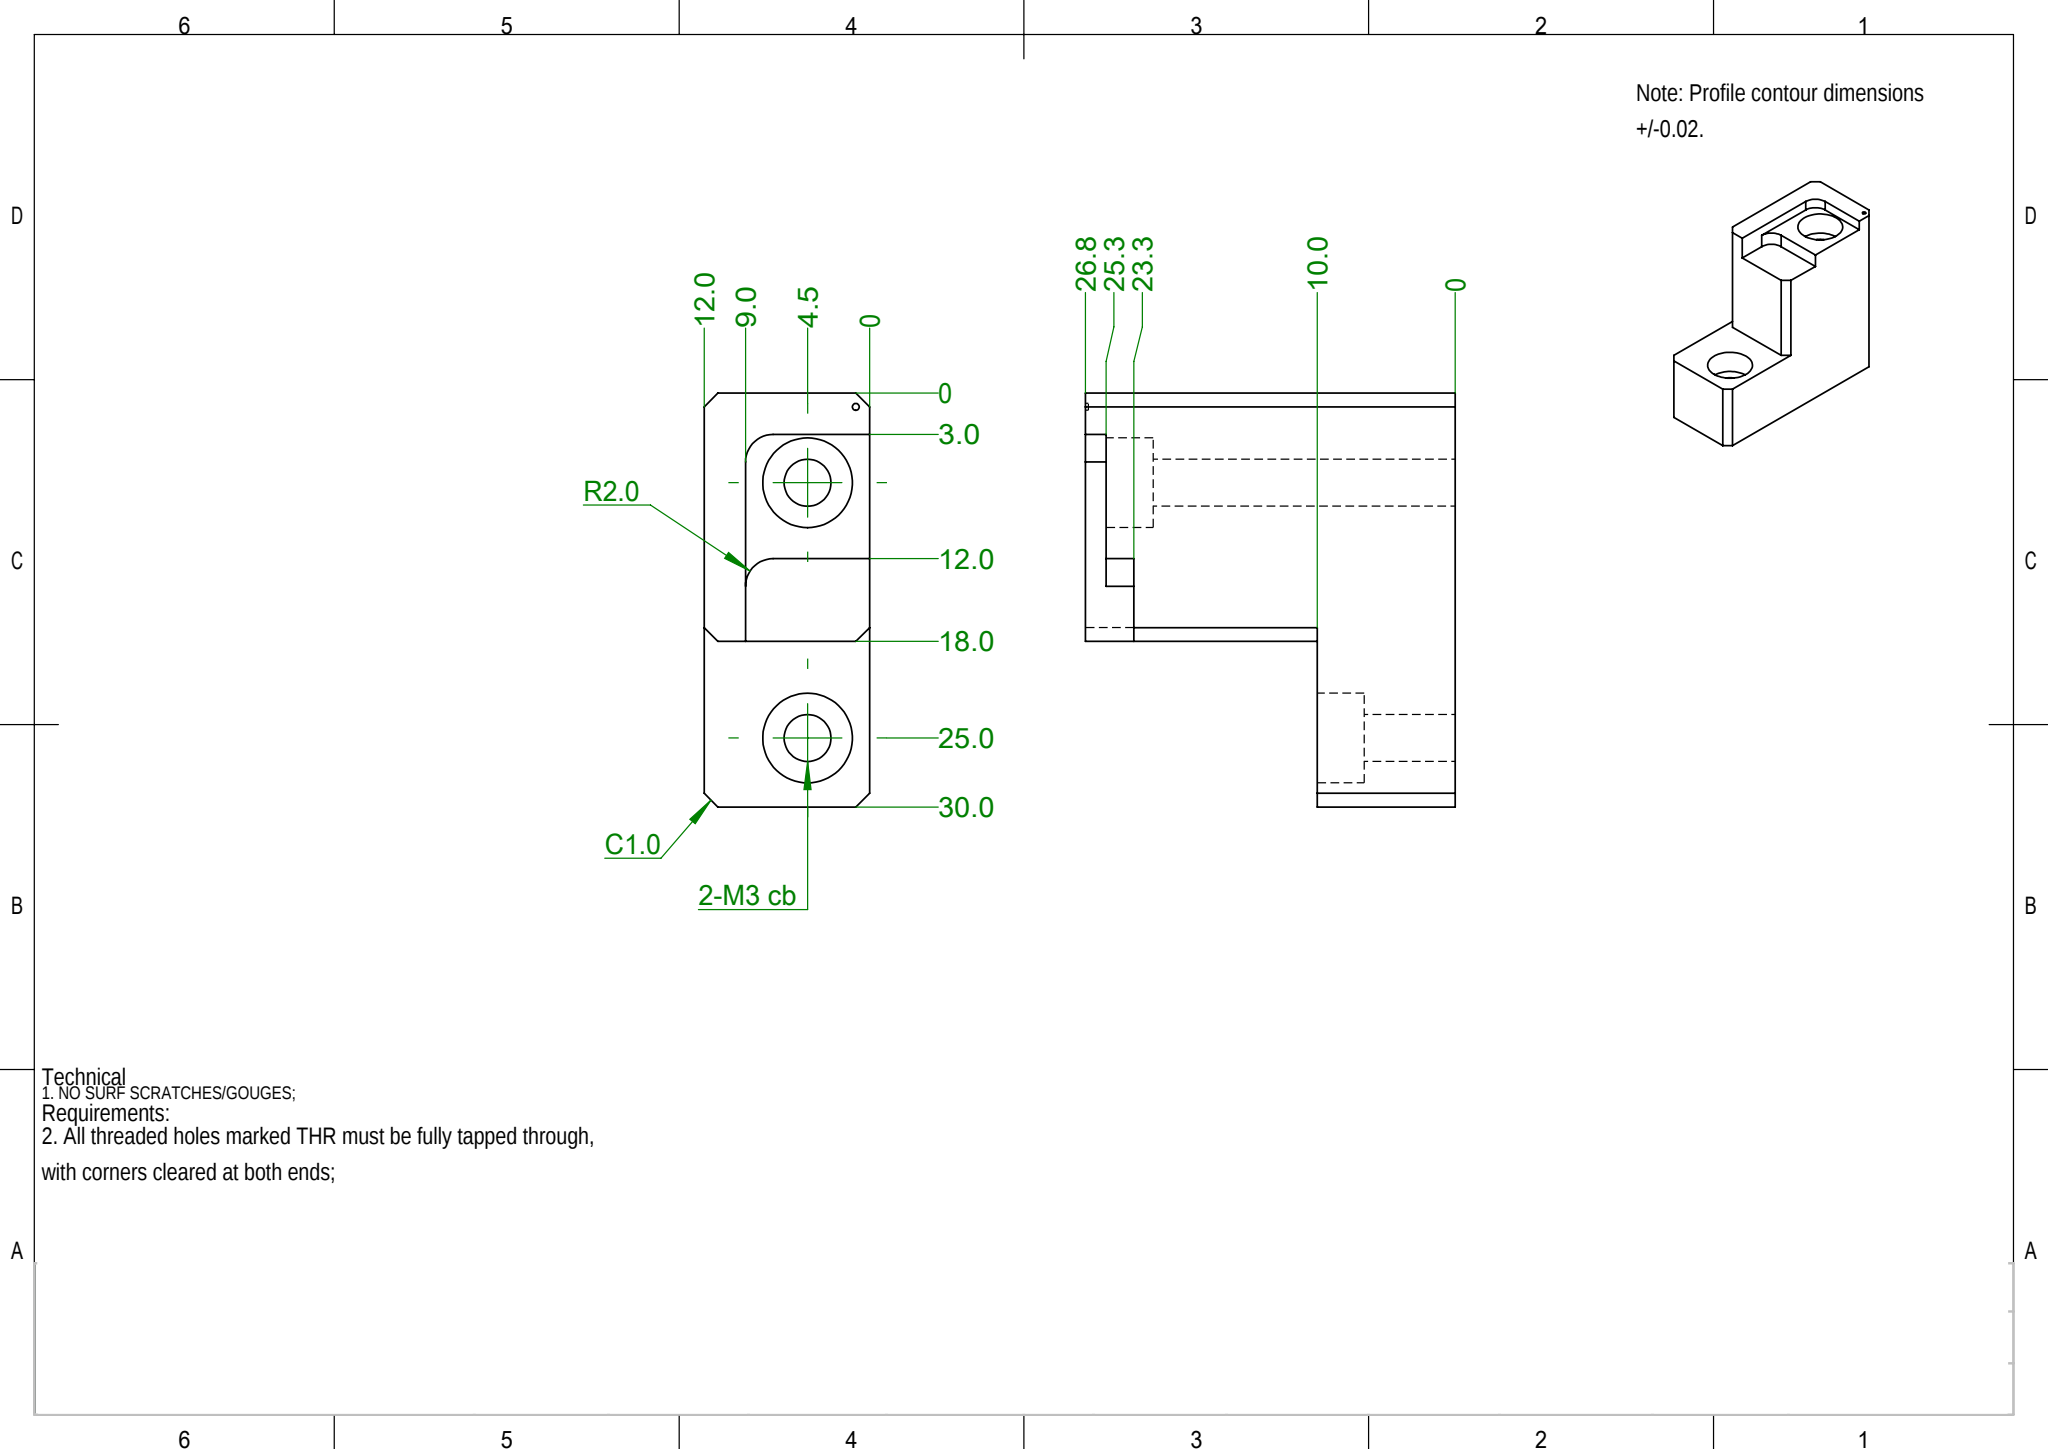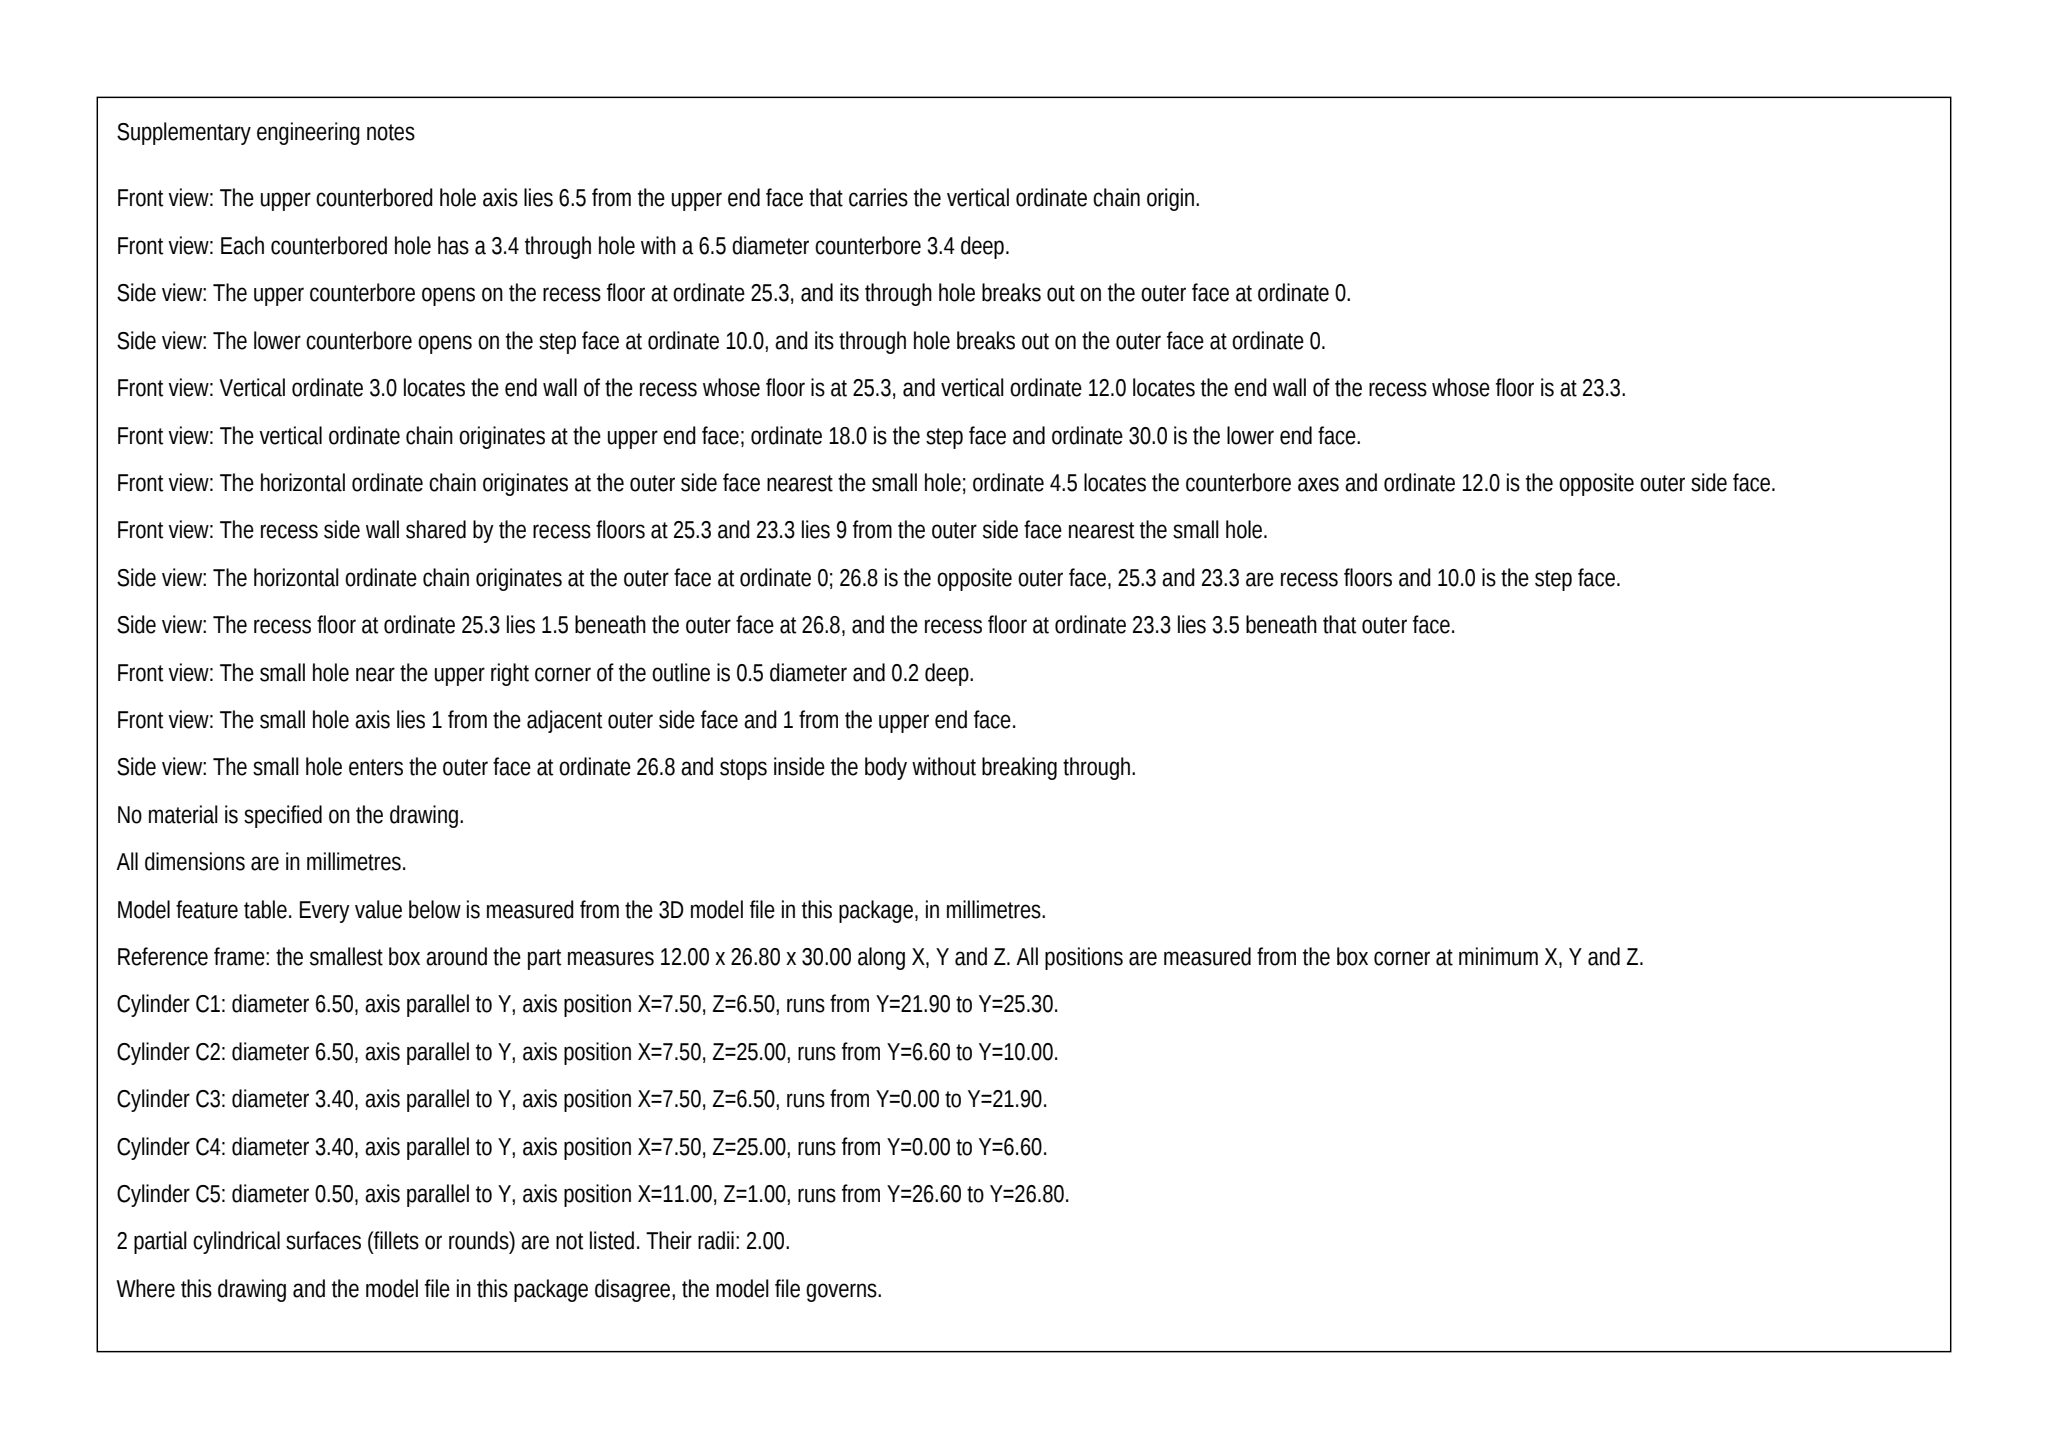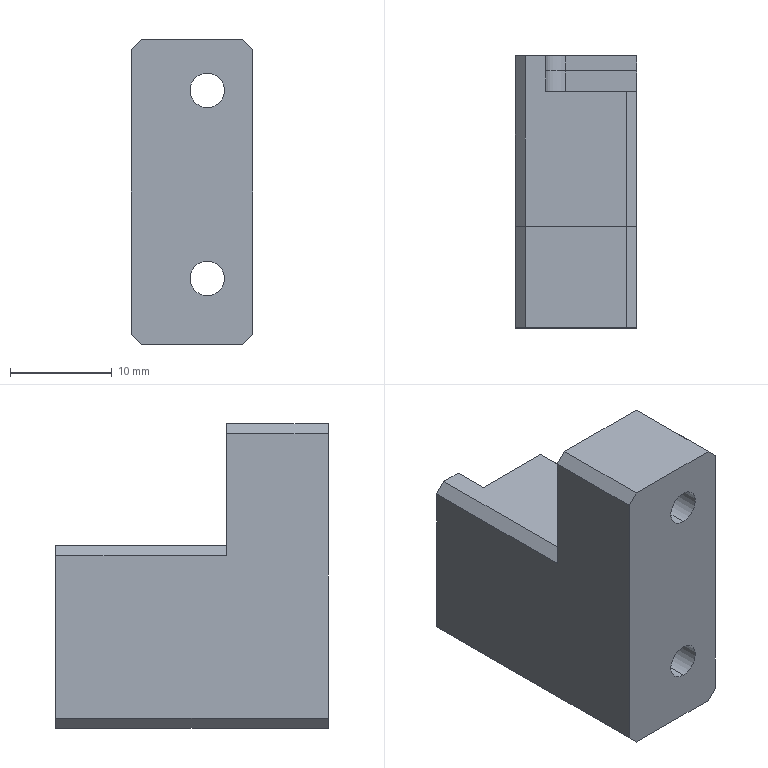Part | SolidWorks | mm | 1 solid | 34 faces | box 12 x 26.8 x 30 mm | volume 6385 mm3 | plane 22 | cylinder 12 | commonest cylinder face diameters 6.5 x4 3.4 x4 0.5 x2 4 x2
Drawing notes:
UPPER M3 CB HOLE CL 6.5 FROM TOP FACE (Z0), X4.5 | from the solid: Ø3.4/Ø6.5 cyls, axis y, pos (x=7.5, z=6.5); bbox X=12 so X ord = 12-7.5 = 4.5; Z from top face = 6.5
2-M3 CB: CBORE Ø6.5 DP 3.4 EA | from the solid: cylinders [6.5,"y",[7.5,-,6.5],3.4] and [6.5,"y",[7.5,-,25.0],3.4]
UPPER CB HOLE: Ø3.4 DP 21.9 BELOW CBORE, THRU TO Y0 FACE | from the solid: cyl [3.4,"y",[7.5,-,6.5],21.9]; cbore btm plane y=25.3-3.4=21.9, drill 21.9 to y=0
LOWER CB HOLE: Ø3.4 DP 6.6 BELOW CBORE, THRU TO Y0 FACE | from the solid: cyl [3.4,"y",[7.5,-,25.0],6.6]; plane y=6.6, leg face y=10.0, 3.4+6.6=10.0
BACK FACE Y0: Ø4.0 DP 1.5 AT Z5.0 & Ø4.0 DP 2.0 AT Z14.0, BOTH X7.0 | from the solid: cyls [4.0,"y",[5.0,-,5.0],1.5] and [4.0,"y",[5.0,-,14.0],2.0]; X ord = 12-5.0 = 7.0
2X Ø0.5 DP 0.2 MARK, X1.0 FROM RH EDGE, Z1.0 FROM TOP | from the solid: cylinders [0.5,"y",[11.0,-,1.0],0.2,2]; X ord = 12-11.0 = 1.0, Z=1.0
FRONT RECESS FACE 0.2 BELOW Y26.8 FACE: ADD ORD Y26.6 | from the solid: axis plane ["y",26.6] vs outer face ["y",26.8]